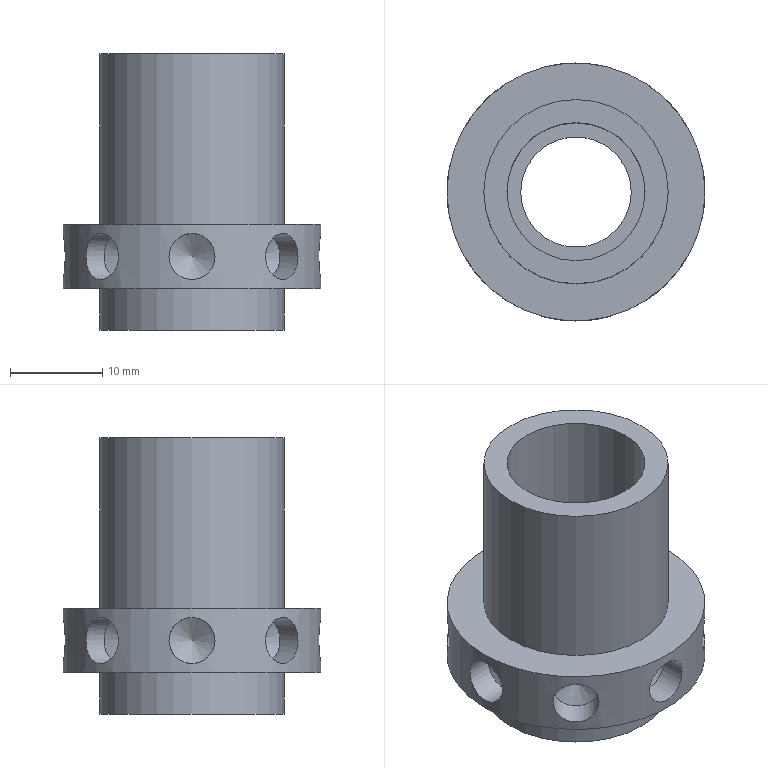Component | NX | EIGHT_HOLE_CLAMP_BLOCK | 1 solid | 26 faces | volume 6015 mm3 | cylinder 13 | cone 8 | plane 5 | commonest cylinder face diameters 5 x8 20 x2 28 x1 15 x1 12 x1